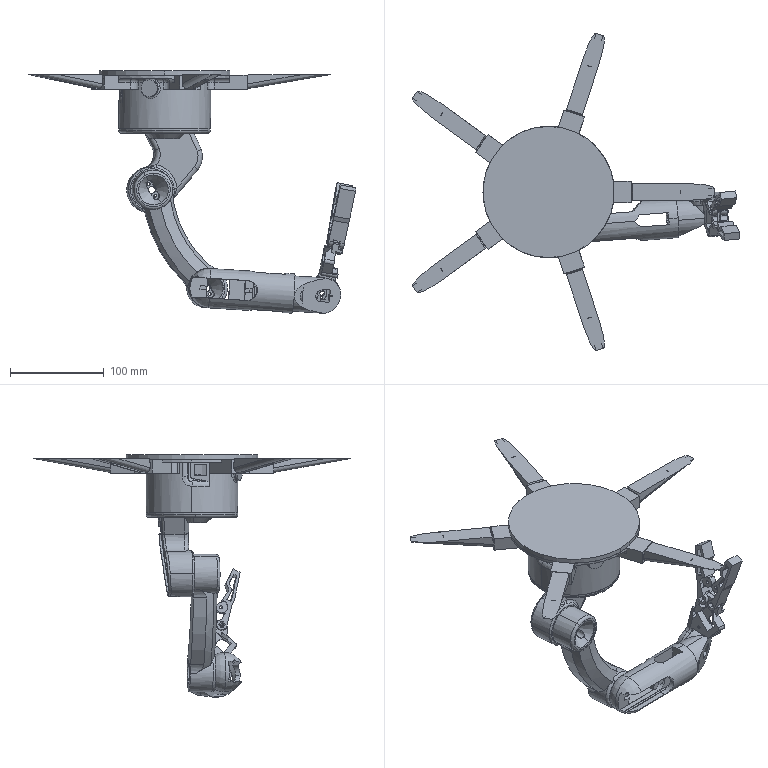Assembly | SolidWorks | mm | 15 component files | 17 solids | 878 faces | box 348.84 x 338.06 x 258.58 mm | volume 612817 mm3 | plane 479 | cylinder 278 | cone 44 | torus 38 | spline 34 | sphere 5 | commonest cylinder face diameters 3 x39 10 x27 16 x13 4.2 x10 6 x10 8 x10 7.5 x10 140 x8
Bill of materials:
Antebrqzo-01-SW | 1 |  | Curved link arm with a round cup-shaped boss at each end. Each cup has a conical recess with a small slotted hole and two small holes at its floor.
Base de la garra-04-SW | 1 |  | Irregular bracket with a flat round disc at one end and a blocky body with stepped plates, a triangular gusset, through holes and a quadrilateral window cutout.
Base-05-SW | 1 |  | Cylindrical sleeve with a wide flat annular flange carrying five radial rectangular tabs. The flange has small holes, and there are inner bosses/brackets and a side round port.
Brazo-06-SW | 1 |  | Elongated hollow tube with a rounded closed end, a narrowed section, and an open or holed opposite end. It has long side slots and rectangular windows.
Cap | 1 |  | Thin flat circular disc with no visible holes or features.
Eje Central-07-SW | 1 |  | Bracket with a flat circular top plate joined by an offset curved arm to a cylindrical hub. The hub has a square through hole.
Mu_eca-10-SW | 1 |  | Hollow housing made from an open cylindrical tube merged with an angled oval-ended block. Its flat face has a rounded-rectangle window, a side slot and a small hole.
Part3 | 1 |  | Solid circular disc, thicker than a thin sheet, with plain faces.
Pata1-11-SW | 1 |  | Elongated tapered blade-like piece with a stepped narrower shank at one end. The far end is rounded/pointed and the cross-section tapers to a thin edge.
Pata2-12-SW | 1 |  | Long wedge-shaped strip with a shoulder step to a narrower shank. One edge tapers to a sharp edge, and the shank end is concave.
Pata3-13-SW | 1 |  | Tapered wedge strip with a stepped shank and a concave end. It looks like a mirrored version of the similar wedge parts.
Pata4-14-SW | 1 |  | Tapered wedge strip with a stepped shoulder, a narrower shank with a rounded end, and a long taper to a thin edge.
Pata5-15-SW | 1 |  | Long, slender, flat bar that tapers to a sharp wedge point in side view. A stepped shoulder block sits near the thick end, then a narrower straight tang ends in a concave curved end face. In plan view it is a strip with one rounded or angled end and a transverse step line.
Pinza1-16-SW | 1 |  | Flat, plate-like lever or link with an irregular zig-zag outline and an enclosed, roughly triangular through-window. One end is a solid rectangular block. The other end has two round eye lugs with through-holes, arranged as a slotted fork.
Pinza2-17-SW | 1 |  | Flat lever or link plate very similar to the other lever part (unnamed part): zig-zag outline, enclosed triangular through-window, solid rectangular block at one end, and two round eye lugs with through-holes forming a slotted fork at the other end. Its features appear on the opposite side from that part, so it may be a mirrored version.
Mates:
1. coincident | Base-05-SW-1 face at (-177.412, -12.412, 1053) dir (0, 0, -1) | Pata1-11-SW-1 face at (-49.274, -27.912, 1053) dir (0, 0, 1)
2. tangent | Base-05-SW-1 edge at (-99.458, -18.912, 1053) dir (0, 0, -1) r 49 | Pata1-11-SW-1 face at (-98.458, -18.912, 1049) dir (0, 0, -1) r 50
3. coincident | Base-05-SW-1 face at (-177.412, -9.912, 1053) dir (0, -1, 0) | Pata1-11-SW-1 face at (76.926, -9.912, 1057.75) dir (0, 1, 0)
4. coincident | Base-05-SW-1 face at (-123.983, 85.696, 1053) dir (-0.9511, -0.309, 0) | Pata4-14-SW-1 face at (-36.393, -183.881, 1057.75) dir (0.9511, 0.309, 0)
5. coincident | Base-05-SW-1 face at (-126.361, 84.923, 1053) dir (0, 0, -1) | Pata4-14-SW-1 face at (-92.51, -69.42, 1053) dir (0, 0, 1)
6. coincident | Base-05-SW-1 face at (-123.983, 85.696, 1053) dir (-0.9511, -0.309, 0) | Pata4-14-SW-1 face at (-36.393, -183.881, 1057.75) dir (0.9511, 0.309, 0)
7. tangent | Base-05-SW-1 face at (-99.458, -18.912, 1000) dir (0, 0, 1) r 49 | Pata4-14-SW-1 face at (-99.149, -19.863, 1049) dir (0, 0, -1) r 50
8. coincident | Base-05-SW-1 face at (4.919, 45.797, 1053) dir (-0.5878, 0.809, 0) | Pata3-13-SW-1 face at (-236.865, -129.868, 1057.75) dir (0.5878, -0.809, 0)
9. coincident | Base-05-SW-1 face at (3.449, 47.82, 1053) dir (0, 0, -1) | Pata3-13-SW-1 face at (-145.347, -41.128, 1053) dir (0, 0, 1)
10. tangent | Base-05-SW-1 face at (-99.458, -18.912, 1000) dir (0, 0, 1) r 49 | Pata3-13-SW-1 face at (-100.267, -19.5, 1049) dir (0, 0, -1) r 50
11. coincident | Base-05-SW-1 face at (-4.192, -96.161, 1053) dir (0, 0, -1) | Pata5-15-SW-1 face at (-134.767, 17.866, 1053) dir (0, 0, 1)
12. coincident | Base-05-SW-1 face at (-5.661, -98.183, 1053) dir (0.5878, 0.809, 0) | Pata5-15-SW-1 face at (-247.445, 77.483, 1057.75) dir (-0.5878, -0.809, 0)
13. tangent | Base-05-SW-1 face at (-99.458, -18.912, 1000) dir (0, 0, 1) r 49 | Pata5-15-SW-1 face at (-100.267, -18.324, 1049) dir (0, 0, -1) r 50
14. coincident | Base-05-SW-1 face at (-138.725, -118.73, 1053) dir (0, 0, -1) | Pata2-12-SW-1 face at (-75.391, 26.034, 1053) dir (0, 0, 1)
15. coincident | Base-05-SW-1 face at (-141.102, -117.957, 1053) dir (0.9511, -0.309, 0) | Pata2-12-SW-1 face at (-53.512, 151.62, 1057.75) dir (-0.9511, 0.309, 0)
16. tangent | Base-05-SW-1 face at (-99.458, -18.912, 1000) dir (0, 0, 1) r 49 | Pata2-12-SW-1 face at (-99.149, -17.961, 1049) dir (0, 0, -1) r 50
17. coincident | Base-05-SW-1 face at (-99.458, -18.912, 1000) dir (0, 0, -1) | Eje Central-07-SW-1 face at (-99.458, -18.912, 1000) dir (0, 0, 1)
18. concentric | Base-05-SW-1 face at (-99.458, -18.912, 1056.75) dir (0, 0, -1) r 46 | Eje Central-07-SW-1 face at (-99.458, -18.912, 995) dir (0, 0, 1) r 49
19. concentric | Eje Central-07-SW-1 face at (-116.043, 13.912, 934.7) dir (0.07679, -0.997, 0) r 24.5 | Antebrqzo-01-SW-1 face at (-113.432, -19.988, 934.7) dir (0.07679, -0.997, 0) r 21
20. coincident | Eje Central-07-SW-1 face at (-123.762, -20.784, 972.691) dir (0.07679, -0.997, 0) | Antebrqzo-01-SW-1 face at (-45.726, -14.773, 938.268) dir (-0.07679, 0.997, 0)
21. coincident | Antebrqzo-01-SW-1 face at (-95.685, -46.203, 998.904) dir (0.07679, -0.997, 0) | Brazo-06-SW-1 face at (-13.697, -39.888, 771.82) dir (-0.07679, 0.997, 0)
22. concentric | Antebrqzo-01-SW-1 face at (-55.086, -15.494, 829.935) dir (0.07679, -0.997, 0) r 21 | Brazo-06-SW-1 face at (-52.183, -53.183, 829.935) dir (1, 0, 0) r 21
23. coincident | Brazo-06-SW-1 face at (37.37, -46.285, 824.227) dir (0.995, 0.07664, -0.06342) | Mu_eca-10-SW-1 face at (37.37, -46.285, 824.227) dir (-0.995, -0.07664, 0.06342)
24. concentric | Brazo-06-SW-1 face at (-73.079, -54.792, 831.267) dir (0.995, 0.07664, -0.06342) r 21 | Mu_eca-10-SW-1 face at (88.615, -42.339, 820.961) dir (-0.995, -0.07664, 0.06342) r 19
25. concentric | Mu_eca-10-SW-1 face at (68.419, -25, 824.636) dir (0.0679, -0.9892, -0.13) r 19 | Base de la garra-04-SW-2 face at (68.745, -29.748, 824.012) dir (-0.0679, 0.9892, 0.13) r 19
26. coincident | Mu_eca-10-SW-1 face at (68.745, -29.748, 824.012) dir (-0.0679, 0.9892, 0.13) | Base de la garra-04-SW-2 face at (68.745, -29.748, 824.012) dir (0.0679, -0.9892, -0.13)
27. concentric | Pinza2-17-SW-1 face at (75.294, -50.962, 880.777) dir (0.9784, 0.09154, -0.1855) r 1.749 | Base de la garra-04-SW-2 face at (73.89, -51.094, 881.043) dir (0.9784, 0.09154, -0.1855) r 1.75
28. width | Pinza2-17-SW-1 face at (70.693, -19.48, 845.522) dir (0.9784, 0.09154, -0.1855) | Pinza2-17-SW-1 face at (77.541, -18.839, 844.224) dir (-0.9784, -0.09154, 0.1855) | Base de la garra-04-SW-2 face at (86.756, -49.89, 878.603) dir (0.9784, 0.09154, -0.1855) | Base de la garra-04-SW-2 face at (71.537, -23.799, 846.739) dir (-0.9784, -0.09154, 0.1855)
29. concentric | Pinza1-16-SW-1 face at (90.867, -36.265, 879.382) dir (-0.9784, -0.09154, 0.1855) r 1.749 | Base de la garra-04-SW-2 face at (72.987, -37.937, 882.772) dir (0.9784, 0.09154, -0.1855) r 1.75
30. width | Pinza1-16-SW-1 face at (82.136, -67.324, 844.535) dir (-0.9784, -0.09154, 0.1855) | Pinza1-16-SW-1 face at (75.288, -67.965, 845.833) dir (0.9784, 0.09154, -0.1855) | Base de la garra-04-SW-2 face at (86.756, -49.89, 878.603) dir (0.9784, 0.09154, -0.1855) | Base de la garra-04-SW-2 face at (71.537, -23.799, 846.739) dir (-0.9784, -0.09154, 0.1855)
31. concentric | Base-05-SW-1 edge at (-115.372, -67.891, 1043.05) dir (0.309, 0.9511, 0) r 9 | Part3-1 face at (-115.372, -67.891, 1043.05) dir (-0.309, -0.9511, 0) r 9
32. coincident | Base-05-SW-1 face at (-115.372, -67.891, 1043.05) dir (-0.309, -0.9511, 0) | Part3-1 face at (-115.372, -67.891, 1043.05) dir (0.309, 0.9511, 0)
33. coincident | Base-05-SW-1 face at (-99.458, -18.912, 1056.75) dir (0, 0, 1) | Cap-1 face at (-99.458, -18.912, 1056.75) dir (0, 0, -1)
34. concentric | Base-05-SW-1 face at (-99.458, -18.912, 1056.75) dir (0, 0, -1) r 70 | Cap-1 face at (-99.458, -18.912, 1061.75) dir (0, 0, -1) r 70